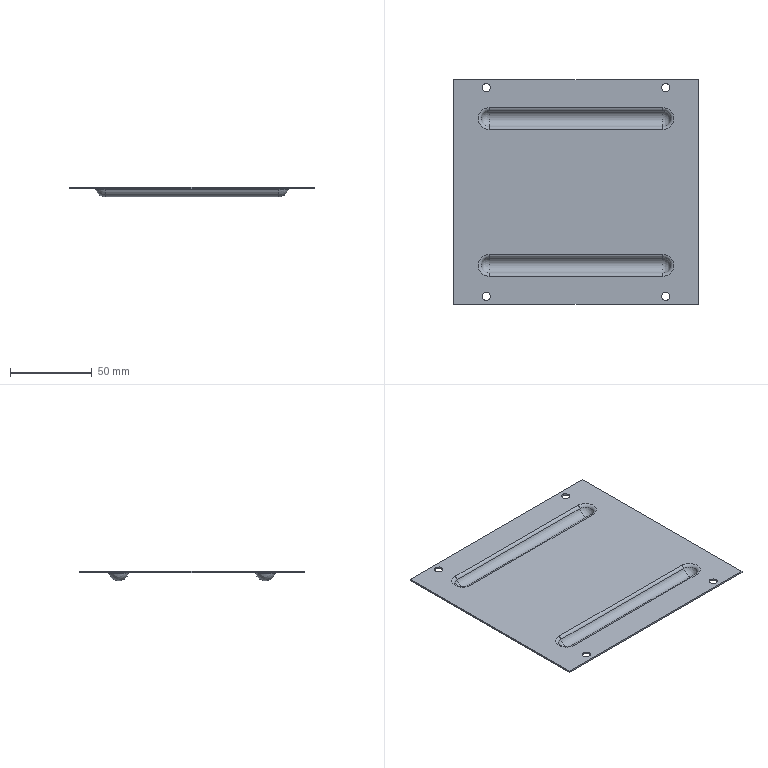Component | NX | TOP_COVER | 1 solid | 38 faces | volume 21715 mm3 | cylinder 16 | sphere 8 | torus 8 | plane 6 | commonest cylinder face diameters 4 x4 2 x4 5 x4 10 x2 12 x2